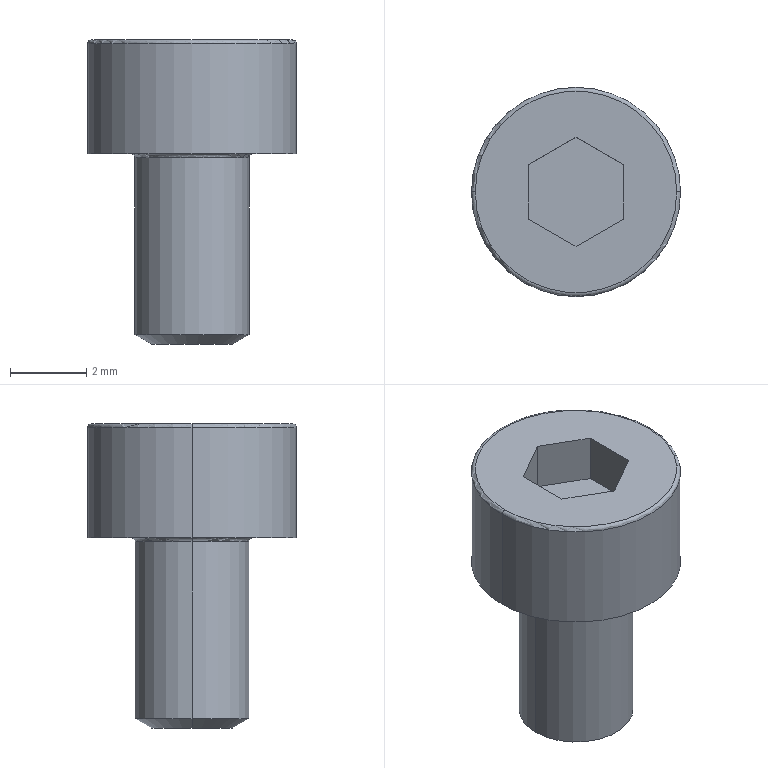Component | NX | GB_T_70_1_2008_HEX_SOCKET_CAP_SCREW_M3X5 | 1 solid | 20 faces | volume 99 mm3 | plane 10 | torus 4 | cylinder 4 | cone 2 | commonest cylinder face diameters 5.5 x2 3 x2